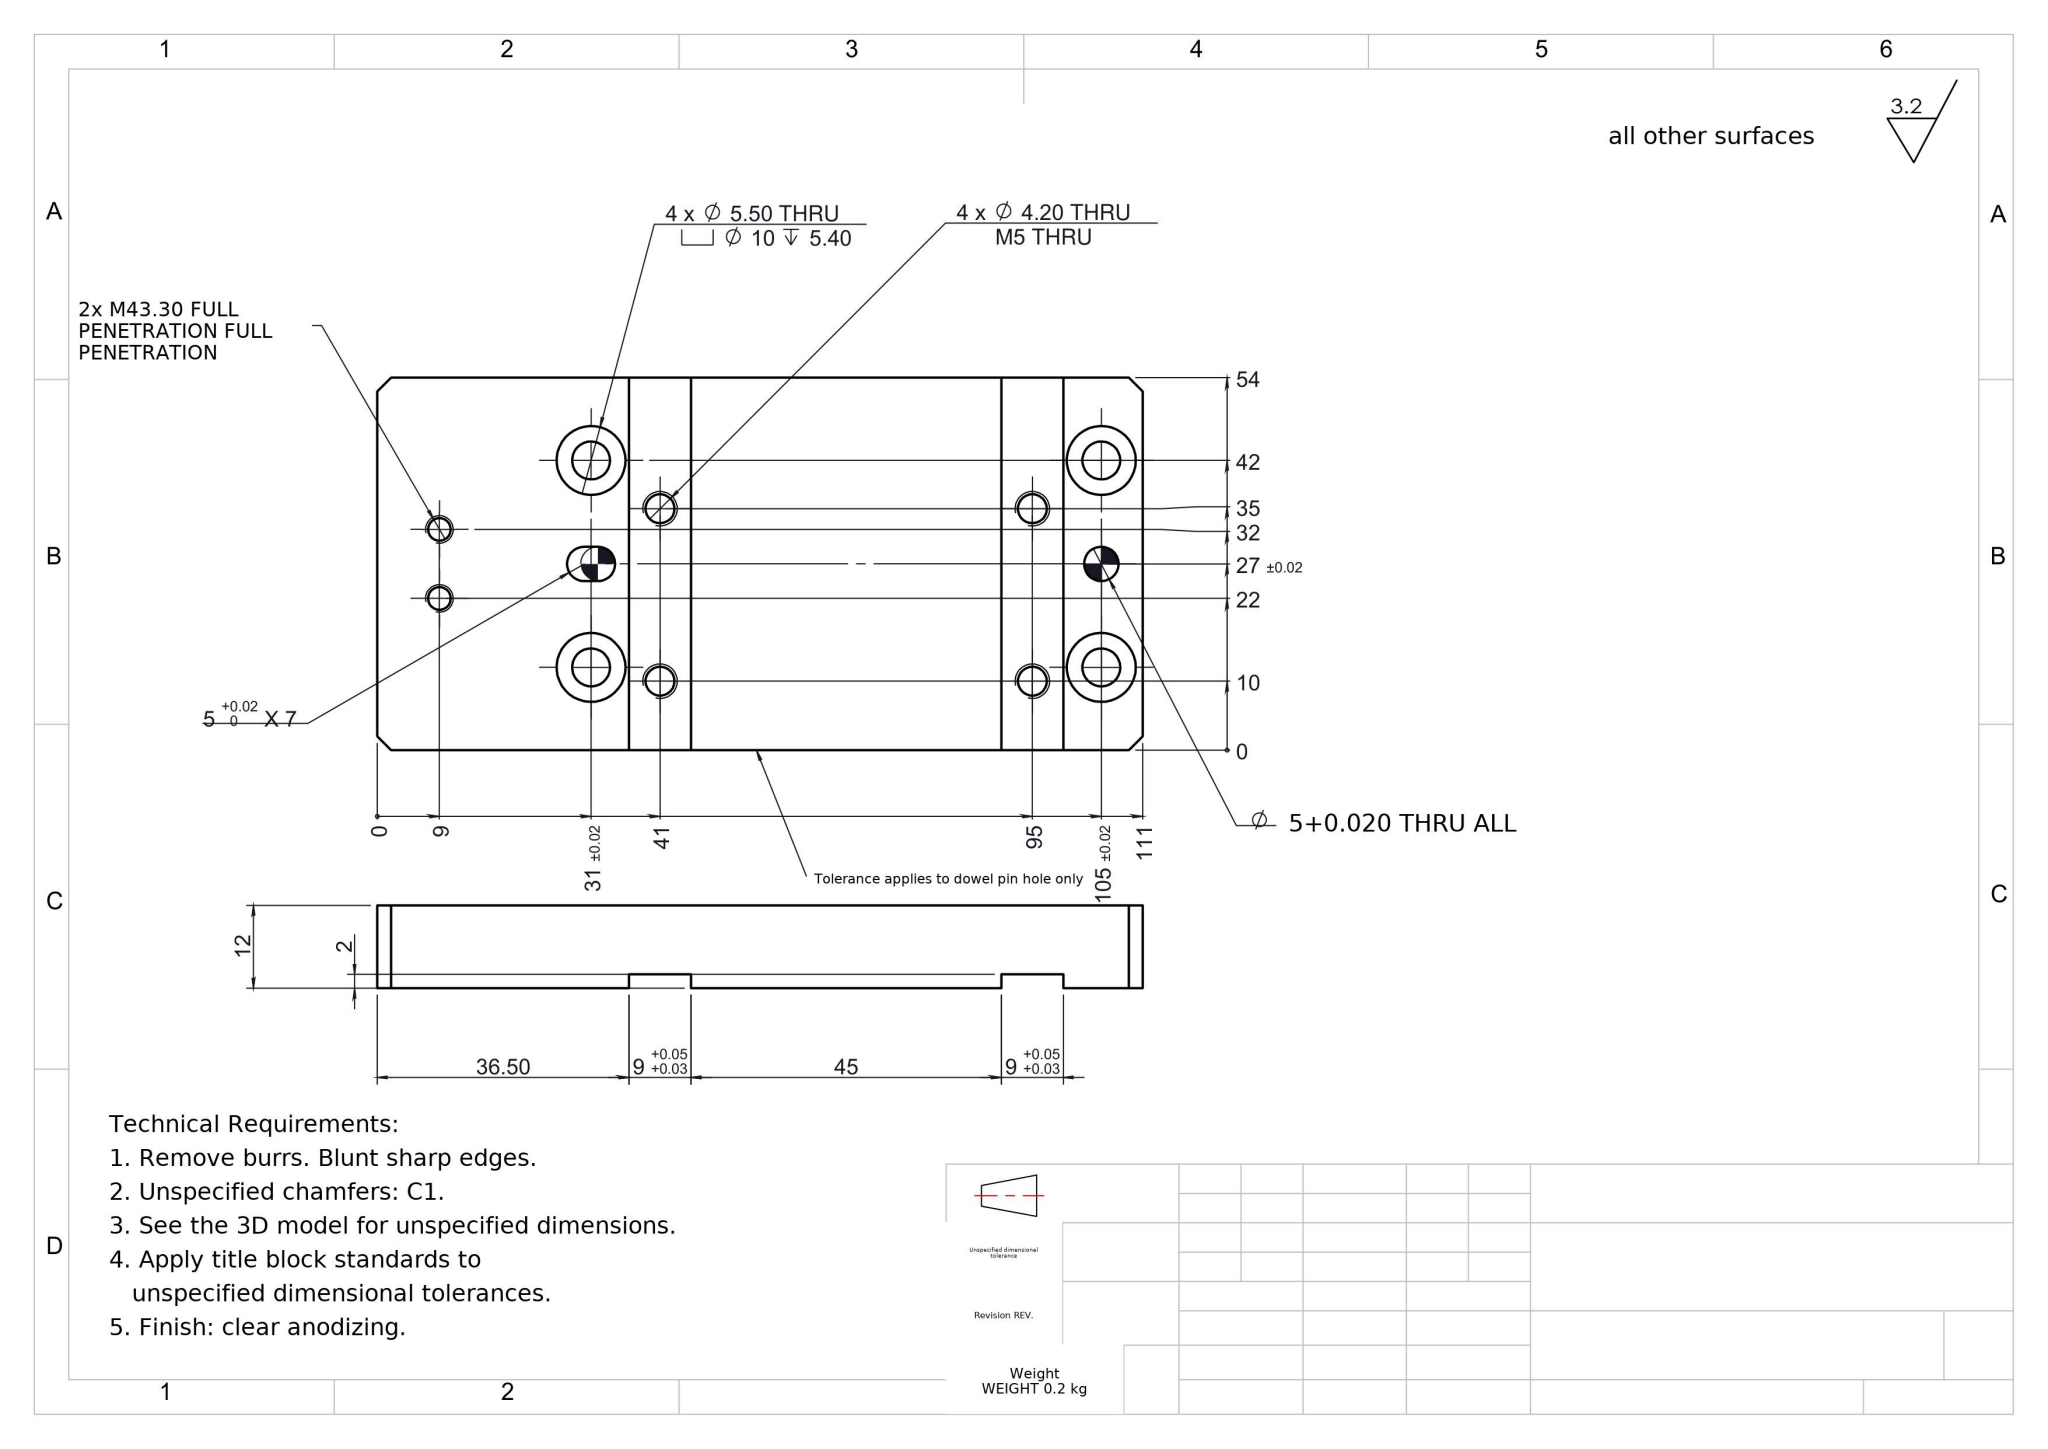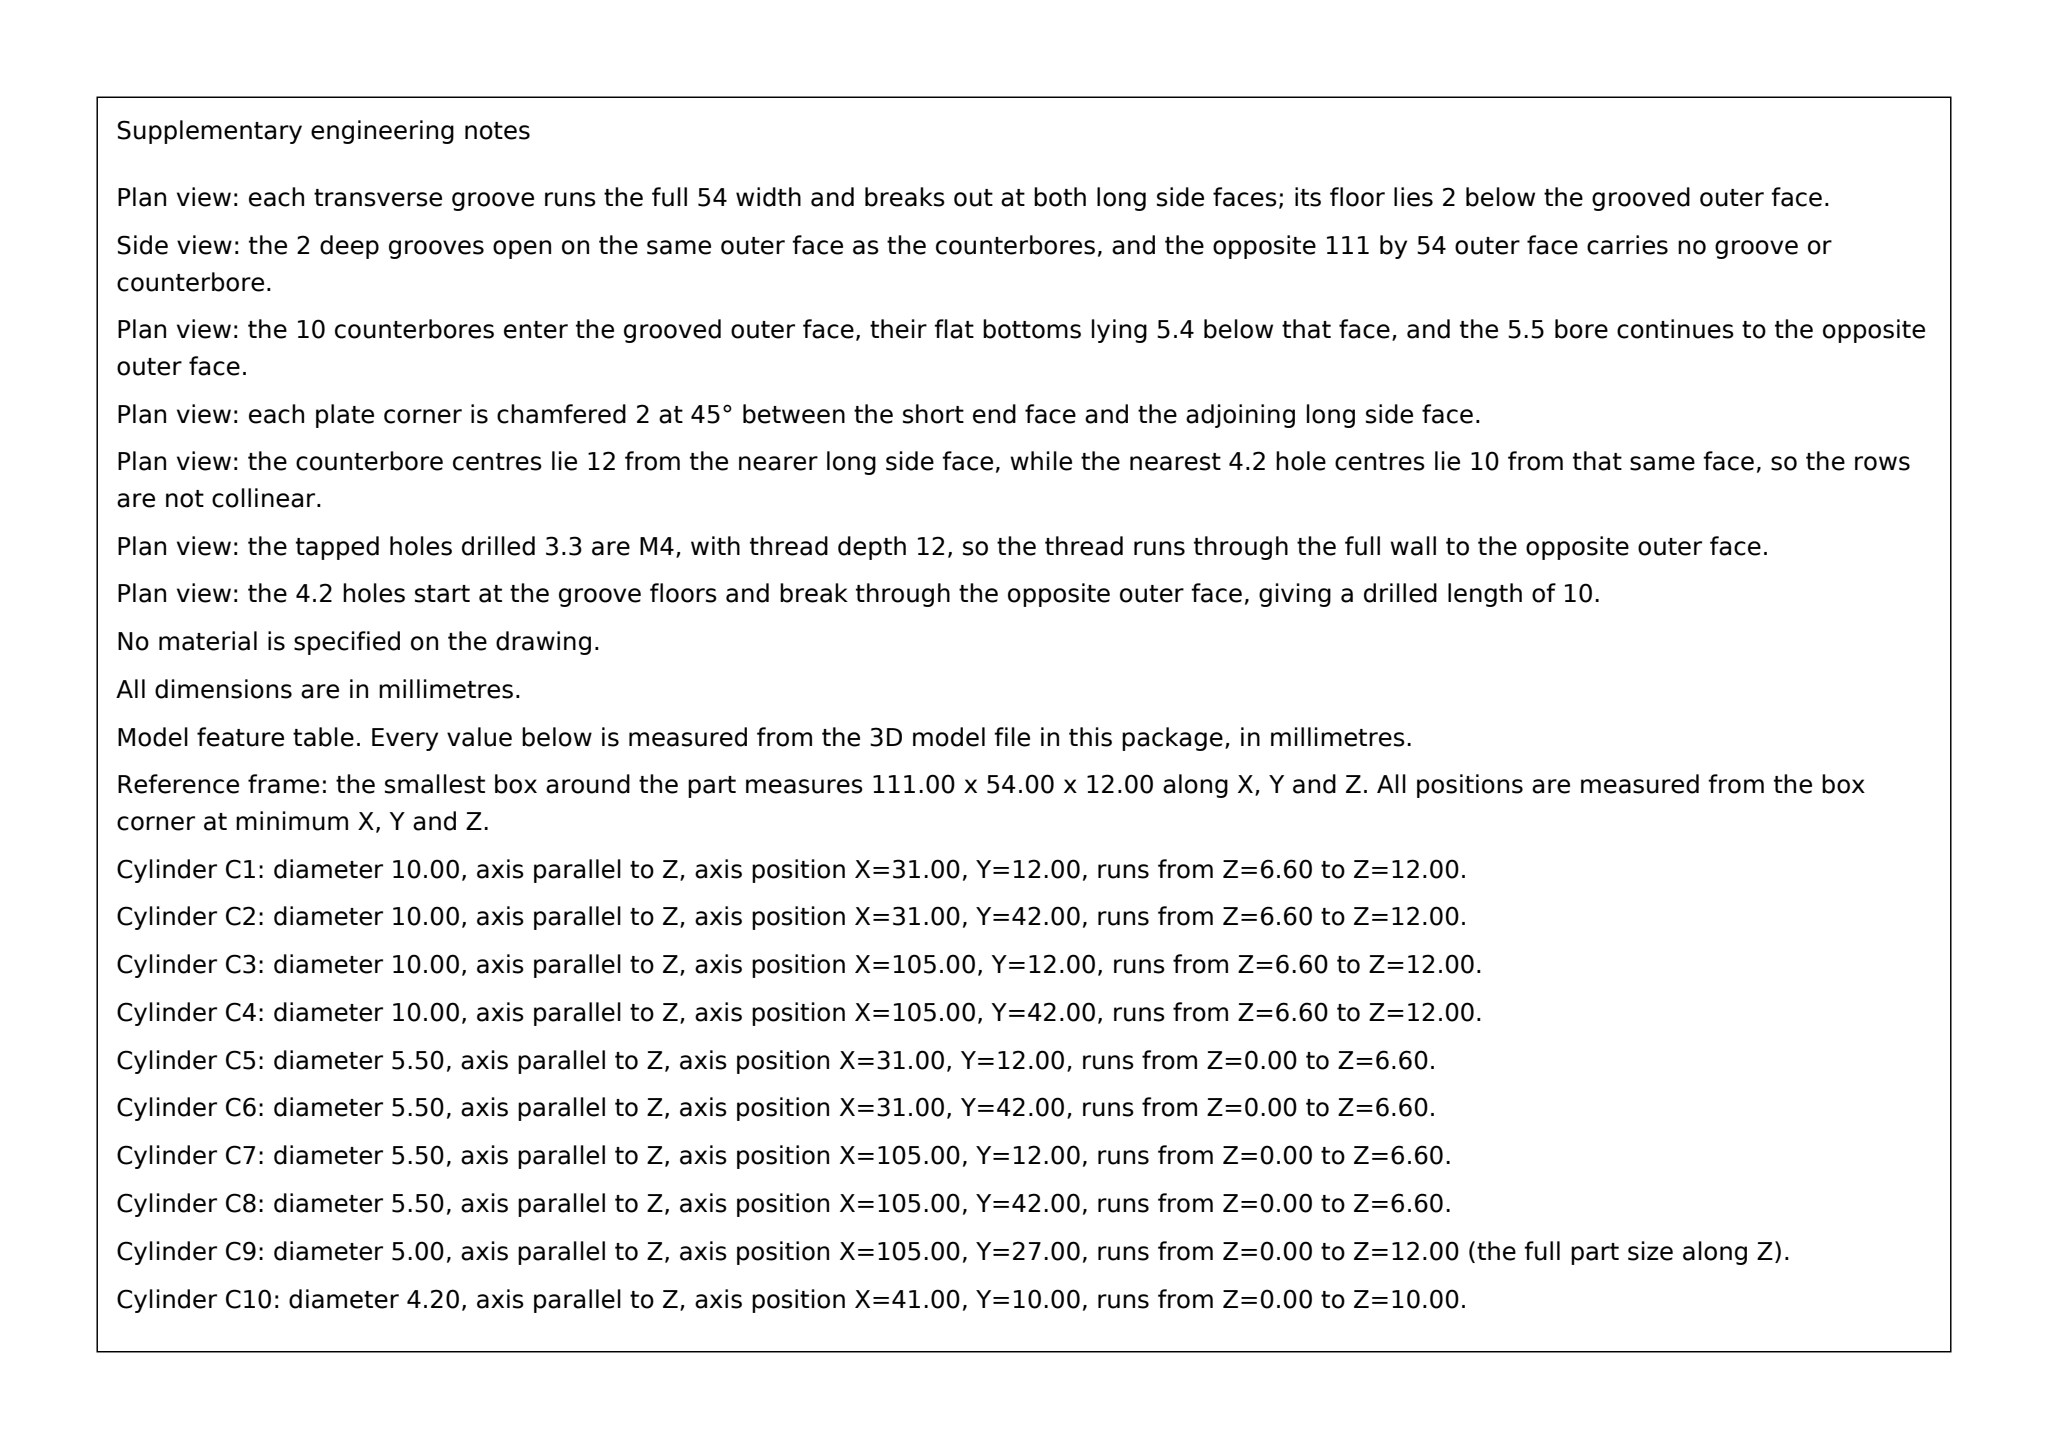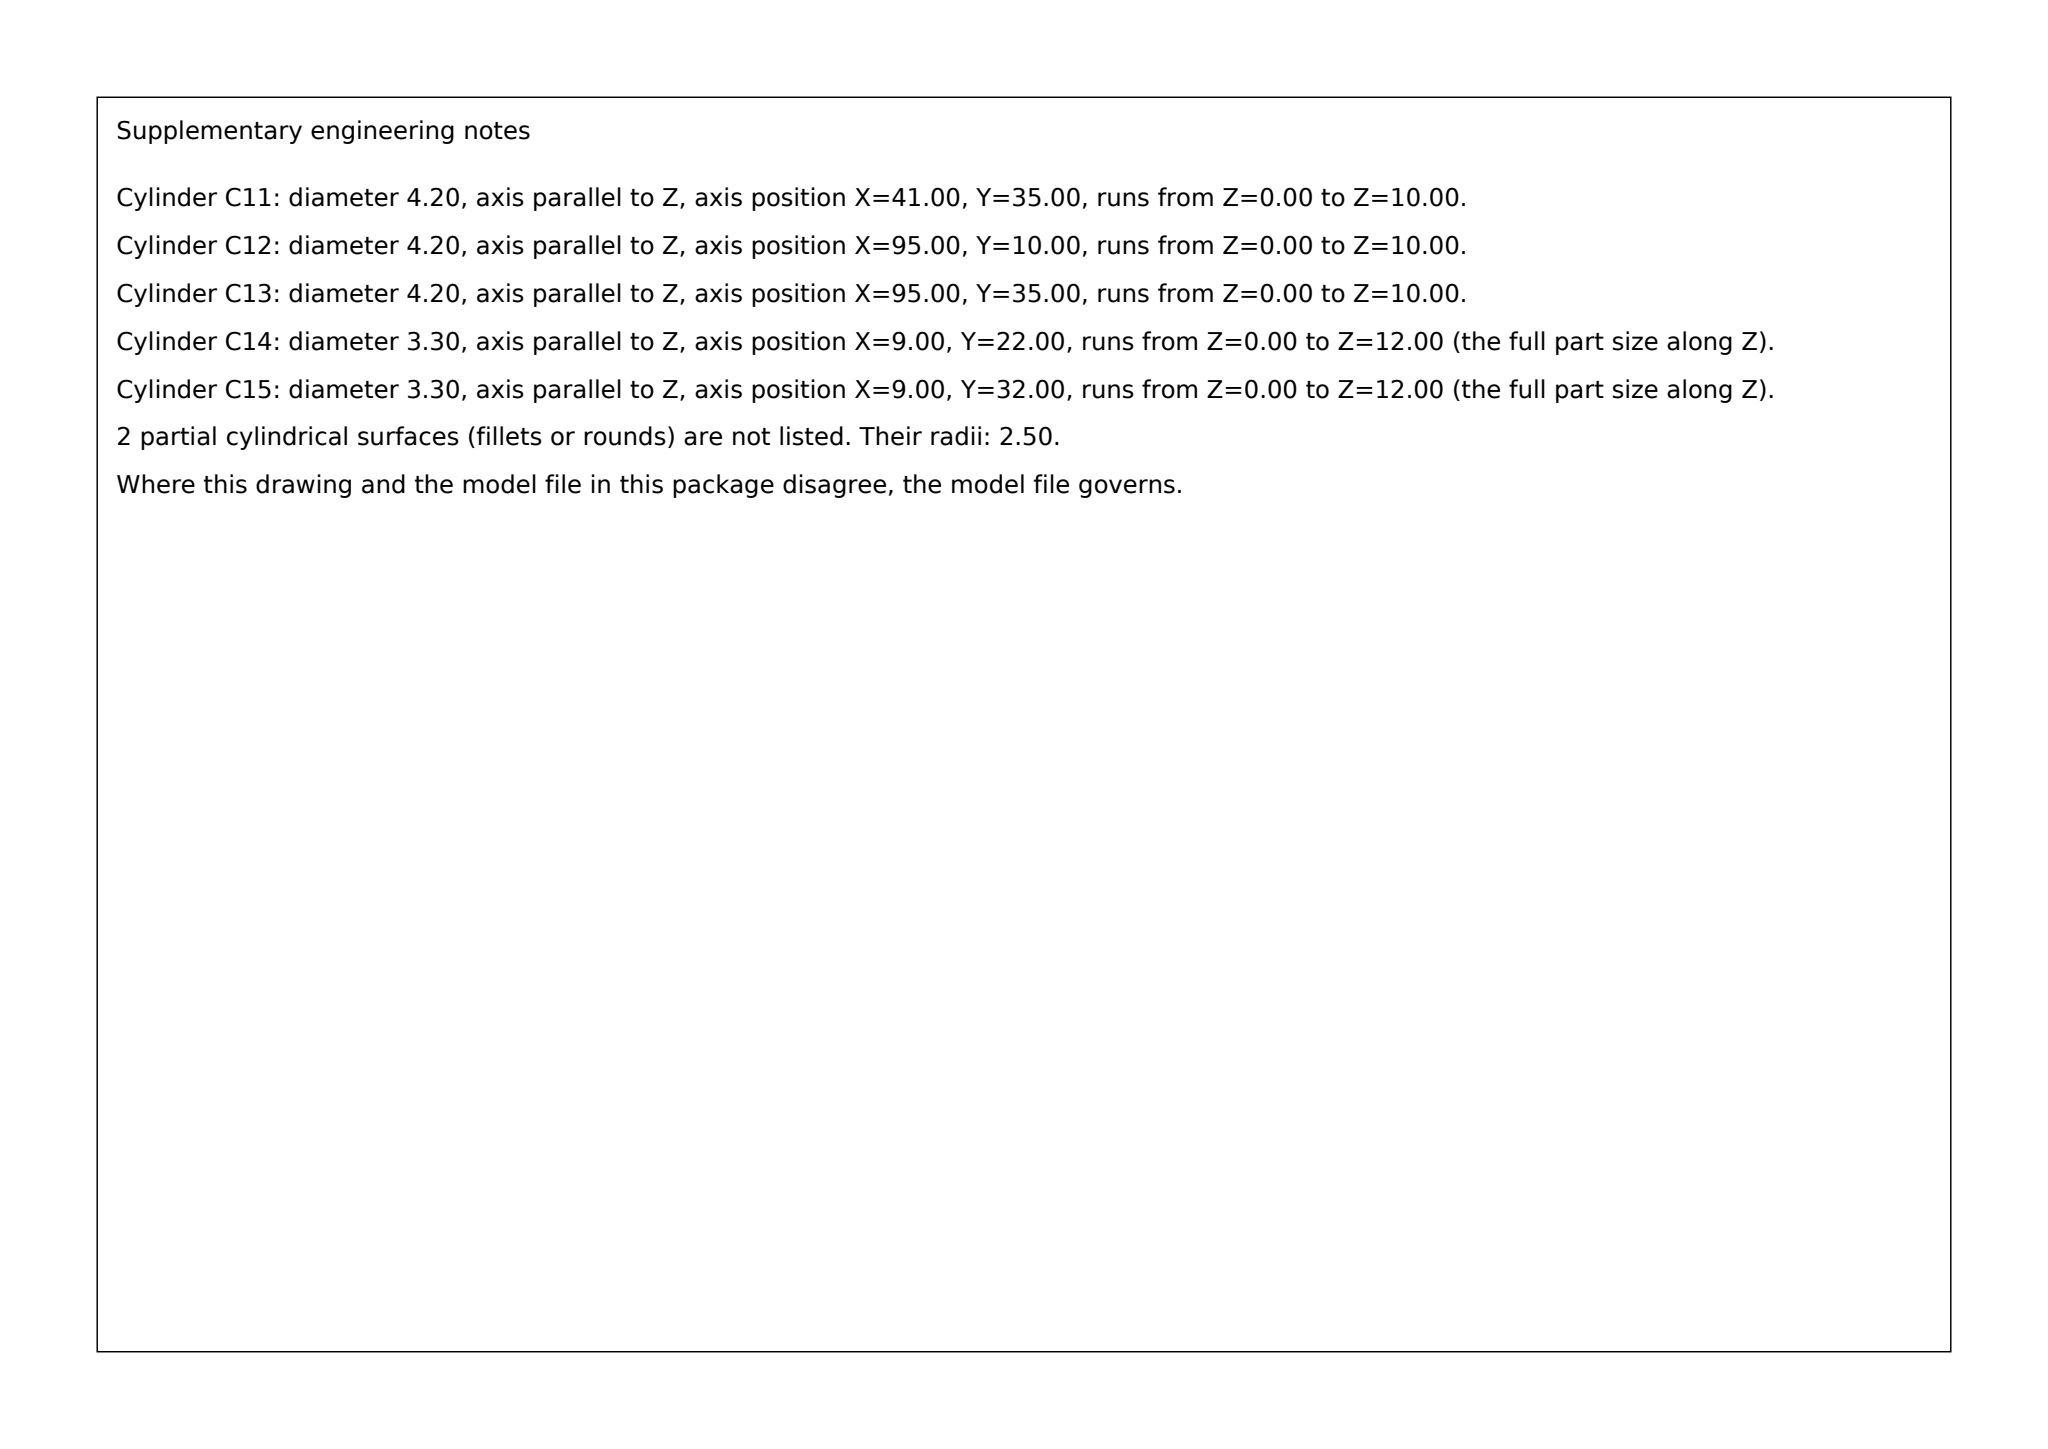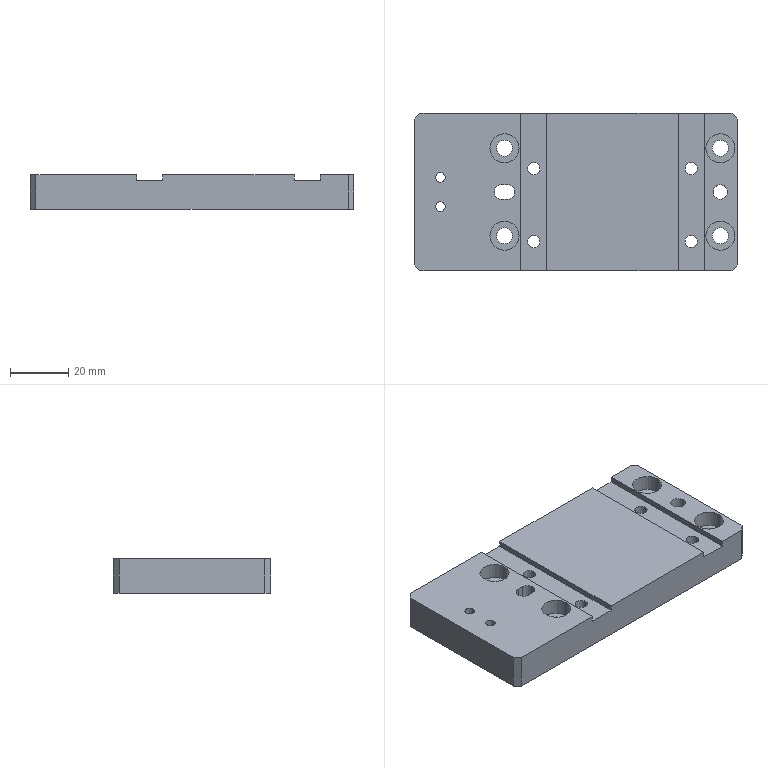Part | SolidWorks | mm | 1 solid | 57 faces | box 111 x 54 x 12 mm | volume 66214 mm3 | cylinder 33 | plane 24 | commonest cylinder face diameters 10 x8 5.5 x8 4.2 x8 5 x5 3.3 x4
Drawing notes:
2X Ø3.30 THRU, M4 THRU (FULL PENETRATION) AT X=9, Y=22 & 32 | from the solid: Ø3.3 z-axis cylinders at (9,22) and (9,32), length 12 = full 12 plate thickness
build123d program:
from build123d import *

# Parameters (mm, degrees)
SKETCH1_W                                       = 86
SKETCH1_H                                       = 54
BOSS_EXTRUDE1_DEPTH                             = 12
SKETCH2_W                                       = 9
SKETCH2_H                                       = 54
CUT_EXTRUDE1_DEPTH                              = 2
M5_TAPPED_HOLE1_D                               = 4.2
M5_HEX_SOCKET_HEAD_CAP_SCREW_CBORE1_D           = 5.5
M5_HEX_SOCKET_HEAD_CAP_SCREW_CBORE1_CBORE_D     = 10
M5_HEX_SOCKET_HEAD_CAP_SCREW_CBORE1_CBORE_DEPTH = 5.4
SIZE_MM_DOWEL_PIN_HOLE1_D                       = 5
SKETCH12_W                                      = 12
SKETCH12_H                                      = 54
BOSS_EXTRUDE4_DEPTH                             = 25
M4_TAPPED_HOLE1_D                               = 3.3
CHAMFER2_SIZE                                   = 2
CUT_EXTRUDE2_DEPTH                              = 75.142


with BuildPart() as part:
    # Sketch1 → Boss-Extrude1 (new body)
    with BuildSketch(Plane.XY):
        Rectangle(SKETCH1_W, SKETCH1_H)
    extrude(amount=BOSS_EXTRUDE1_DEPTH)

    # Sketch2 → Cut-Extrude1 (cut)
    with BuildSketch(Plane.XY.offset(12)):
        with Locations((-27, 0)):
            Rectangle(SKETCH2_W, SKETCH2_H)
        with Locations((27, 0)):
            Rectangle(SKETCH2_W, SKETCH2_H)
    extrude(amount=-CUT_EXTRUDE1_DEPTH, mode=Mode.SUBTRACT)

    # M5 Tapped Hole1 (through all)
    with Locations(Plane.XY.offset(10)):
        with Locations((27, -17), (27, 8), (-27, -17), (-27, 8)):
            Hole(M5_TAPPED_HOLE1_D / 2)

    # M5 Hex Socket Head Cap Screw CBORE1 (through all)
    with Locations(Plane.XY.offset(12)):
        with Locations((-37, -15), (-37, 15), (37, -15), (37, 15)):
            CounterBoreHole(M5_HEX_SOCKET_HEAD_CAP_SCREW_CBORE1_D / 2, M5_HEX_SOCKET_HEAD_CAP_SCREW_CBORE1_CBORE_D / 2, M5_HEX_SOCKET_HEAD_CAP_SCREW_CBORE1_CBORE_DEPTH)

    # Size mm Dowel Pin Hole1 (through all)
    with Locations(Plane.XY.offset(12)):
        with Locations((-37, 0), (37, 0)):
            Hole(SIZE_MM_DOWEL_PIN_HOLE1_D / 2)

    # Sketch12 → Boss-Extrude4 (add)
    with BuildSketch(Plane.ZY.offset(43)):
        with Locations((6, 0)):
            Rectangle(SKETCH12_W, SKETCH12_H)
    extrude(amount=BOSS_EXTRUDE4_DEPTH)

    # M4 Tapped Hole1 (through all)
    with Locations(Plane(origin=(0, 0, 0), x_dir=(-1, 0, 0), z_dir=(0, 0, -1))):
        with Locations((59, -5), (59, 5)):
            Hole(M4_TAPPED_HOLE1_D / 2)

    # Chamfer2
    chamfer2_edges = [part.edges().sort_by_distance(p)[0] for p in [
        (-68, -27, 6),
        (-68, 27, 6),
        (43, -27, 6),
        (43, 27, 6),
    ]]
    chamfer(chamfer2_edges, length=CHAMFER2_SIZE)

    # Sketch15 → Cut-Extrude2 (cut, through all)
    with BuildSketch(Plane.XY.offset(12)):
        with BuildLine():
            Line((-38, 2.5), (-36, 2.5))
            ThreePointArc((-36, 2.5), (-33.5, 0), (-36, -2.5))
            Line((-36, -2.5), (-38, -2.5))
            ThreePointArc((-38, -2.5), (-40.5, 0), (-38, 2.5))
        make_face()
    extrude(amount=-CUT_EXTRUDE2_DEPTH, mode=Mode.SUBTRACT)


solid = part.part